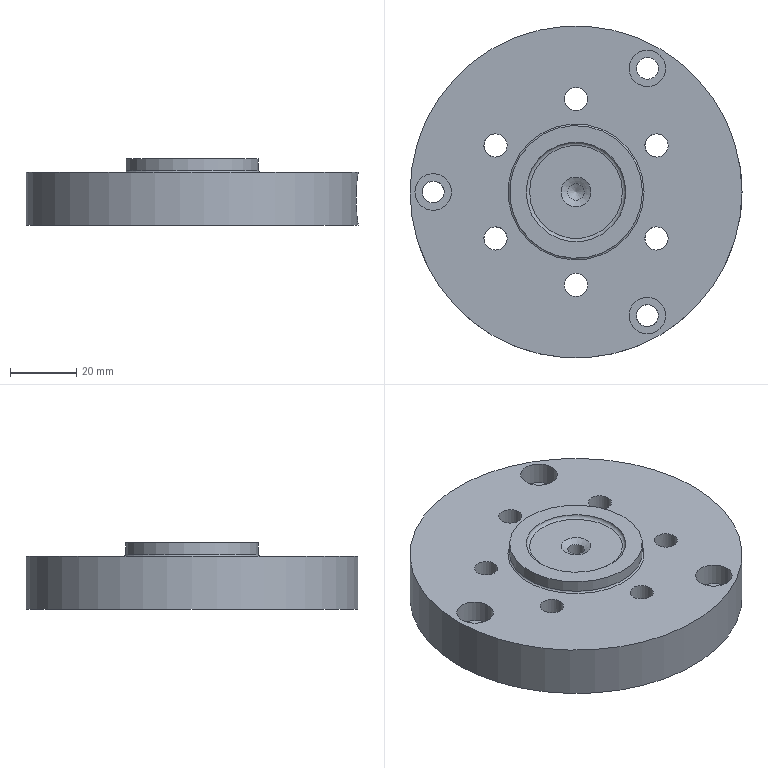Component | NX | END_CAP | 1 solid | 45 faces | volume 115510 mm3 | cylinder 24 | plane 16 | torus 3 | cone 2 | commonest cylinder face diameters 11 x9 7 x6 6.6 x3 5 x2 100 x1 8.56 x1 40 x1 15.2 x1